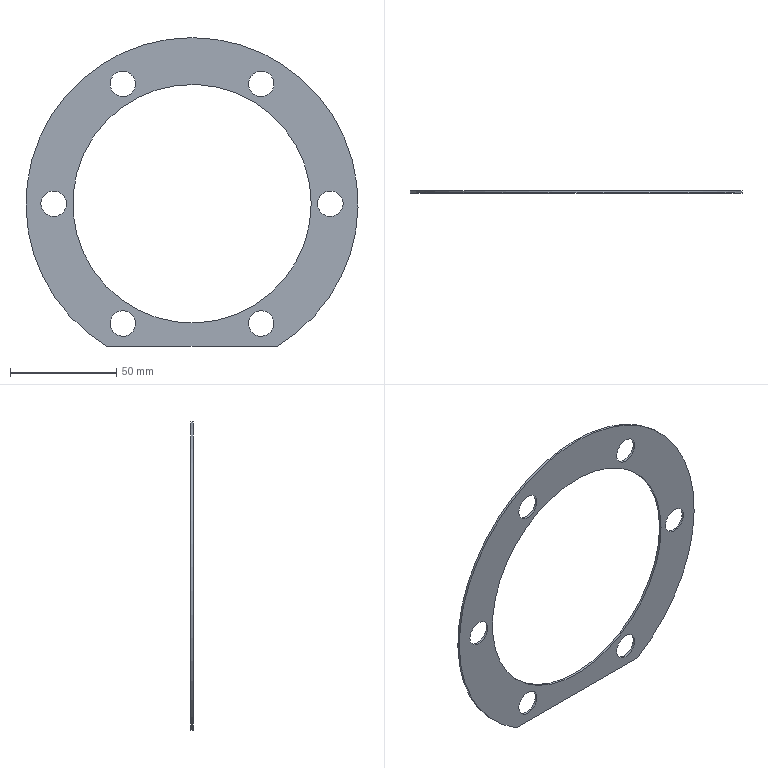Component | NX | T1_SHIM2_2 | 1 solid | 11 faces | box 156 x 1 x 145 mm | volume 7988 mm3 | cylinder 8 | plane 3 | commonest cylinder face diameters 12 x6 156 x1 112 x1
STEP:
#1=CARTESIAN_POINT('',(0.,0.,0.));
#2=DIRECTION('',(0.,0.,1.));
#3=DIRECTION('',(1.,0.,0.));
#4=AXIS2_PLACEMENT_3D('',#1,#2,#3);
#5=CARTESIAN_POINT('',(44.937,28.,198.5));
#6=VERTEX_POINT('',#5);
#7=CARTESIAN_POINT('',(-34.937,28.,198.5));
#8=VERTEX_POINT('',#7);
#9=CARTESIAN_POINT('',(5.,28.,265.5));
#10=DIRECTION('',(0.,-1.,0.));
#11=DIRECTION('',(1.,0.,0.));
#12=AXIS2_PLACEMENT_3D('',#9,#10,#11);
#13=CIRCLE('',#12,78.);
#14=CARTESIAN_POINT('',(5.,27.,265.5));
#15=DIRECTION('',(0.,1.,0.));
#16=DIRECTION('',(-1.,0.,0.));
#17=AXIS2_PLACEMENT_3D('',#14,#15,#16);
#18=CYLINDRICAL_SURFACE('',#17,78.);
#19=CARTESIAN_POINT('',(9.425,1.));
#20=DIRECTION('',(-1.,0.));
#21=VECTOR('',#20,1.);
#22=LINE('',#19,#21);
#23=(GEOMETRIC_REPRESENTATION_CONTEXT(2)PARAMETRIC_REPRESENTATION_CONTEXT()REPRESENTATION_CONTEXT('',''));
#24=DEFINITIONAL_REPRESENTATION('',(#22),#23);
#25=PCURVE('',#18,#24);
#26=CARTESIAN_POINT('',(5.,28.,265.5));
#27=DIRECTION('',(0.,-1.,0.));
#28=DIRECTION('',(1.,0.,0.));
#29=AXIS2_PLACEMENT_3D('',#26,#27,#28);
#30=PLANE('',#29);
#31=CARTESIAN_POINT('',(0.,0.));
#32=DIRECTION('',(1.,0.));
#33=AXIS2_PLACEMENT_2D('',#31,#32);
#34=CIRCLE('',#33,78.);
#35=(GEOMETRIC_REPRESENTATION_CONTEXT(2)PARAMETRIC_REPRESENTATION_CONTEXT()REPRESENTATION_CONTEXT('',''));
#36=DEFINITIONAL_REPRESENTATION('',(#34),#35);
#37=PCURVE('',#30,#36);
#38=SURFACE_CURVE('',#13,(#25,#37),.PCURVE_S1.);
#39=EDGE_CURVE('',#6,#8,#38,.T.);
#40=ORIENTED_EDGE('',*,*,#39,.T.);
#41=CARTESIAN_POINT('',(-34.937,27.,198.5));
#42=VERTEX_POINT('',#41);
#43=CARTESIAN_POINT('',(-34.937,27.,198.5));
#44=DIRECTION('',(0.,1.,0.));
#45=VECTOR('',#44,1.);
#46=LINE('',#43,#45);
#47=CARTESIAN_POINT('',(-1.033,0.));
#48=DIRECTION('',(0.,1.));
#49=VECTOR('',#48,1.);
#50=LINE('',#47,#49);
#51=(GEOMETRIC_REPRESENTATION_CONTEXT(2)PARAMETRIC_REPRESENTATION_CONTEXT()REPRESENTATION_CONTEXT('',''));
#52=DEFINITIONAL_REPRESENTATION('',(#50),#51);
#53=PCURVE('',#18,#52);
#54=CARTESIAN_POINT('',(-34.937,27.,198.5));
#55=DIRECTION('',(0.,0.,1.));
#56=DIRECTION('',(0.,-1.,0.));
#57=AXIS2_PLACEMENT_3D('',#54,#55,#56);
#58=PLANE('',#57);
#59=CARTESIAN_POINT('',(0.,0.));
#60=DIRECTION('',(-1.,0.));
#61=VECTOR('',#60,1.);
#62=LINE('',#59,#61);
#63=(GEOMETRIC_REPRESENTATION_CONTEXT(2)PARAMETRIC_REPRESENTATION_CONTEXT()REPRESENTATION_CONTEXT('',''));
#64=DEFINITIONAL_REPRESENTATION('',(#62),#63);
#65=PCURVE('',#58,#64);
#66=SURFACE_CURVE('',#46,(#53,#65),.PCURVE_S1.);
#67=EDGE_CURVE('',#42,#8,#66,.T.);
#68=ORIENTED_EDGE('',*,*,#67,.F.);
#69=CARTESIAN_POINT('',(44.937,27.,198.5));
#70=VERTEX_POINT('',#69);
#71=CARTESIAN_POINT('',(5.,27.,265.5));
#72=DIRECTION('',(0.,-1.,0.));
#73=DIRECTION('',(1.,0.,0.));
#74=AXIS2_PLACEMENT_3D('',#71,#72,#73);
#75=CIRCLE('',#74,78.);
#76=CARTESIAN_POINT('',(9.425,0.));
#77=DIRECTION('',(-1.,0.));
#78=VECTOR('',#77,1.);
#79=LINE('',#76,#78);
#80=(GEOMETRIC_REPRESENTATION_CONTEXT(2)PARAMETRIC_REPRESENTATION_CONTEXT()REPRESENTATION_CONTEXT('',''));
#81=DEFINITIONAL_REPRESENTATION('',(#79),#80);
#82=PCURVE('',#18,#81);
#83=CARTESIAN_POINT('',(5.,27.,265.5));
#84=DIRECTION('',(0.,-1.,0.));
#85=DIRECTION('',(1.,0.,0.));
#86=AXIS2_PLACEMENT_3D('',#83,#84,#85);
#87=PLANE('',#86);
#88=CARTESIAN_POINT('',(0.,0.));
#89=DIRECTION('',(1.,0.));
#90=AXIS2_PLACEMENT_2D('',#88,#89);
#91=CIRCLE('',#90,78.);
#92=(GEOMETRIC_REPRESENTATION_CONTEXT(2)PARAMETRIC_REPRESENTATION_CONTEXT()REPRESENTATION_CONTEXT('',''));
#93=DEFINITIONAL_REPRESENTATION('',(#91),#92);
#94=PCURVE('',#87,#93);
#95=SURFACE_CURVE('',#75,(#82,#94),.PCURVE_S1.);
#96=EDGE_CURVE('',#70,#42,#95,.T.);
#97=ORIENTED_EDGE('',*,*,#96,.F.);
#98=CARTESIAN_POINT('',(44.937,27.,198.5));
#99=DIRECTION('',(0.,-1.,0.));
#100=VECTOR('',#99,1.);
#101=LINE('',#98,#100);
#102=CARTESIAN_POINT('',(4.175,0.));
#103=DIRECTION('',(0.,-1.));
#104=VECTOR('',#103,1.);
#105=LINE('',#102,#104);
#106=(GEOMETRIC_REPRESENTATION_CONTEXT(2)PARAMETRIC_REPRESENTATION_CONTEXT()REPRESENTATION_CONTEXT('',''));
#107=DEFINITIONAL_REPRESENTATION('',(#105),#106);
#108=PCURVE('',#18,#107);
#109=CARTESIAN_POINT('',(0.,79.875));
#110=DIRECTION('',(1.,0.));
#111=VECTOR('',#110,1.);
#112=LINE('',#109,#111);
#113=(GEOMETRIC_REPRESENTATION_CONTEXT(2)PARAMETRIC_REPRESENTATION_CONTEXT()REPRESENTATION_CONTEXT('',''));
#114=DEFINITIONAL_REPRESENTATION('',(#112),#113);
#115=PCURVE('',#58,#114);
#116=SURFACE_CURVE('',#101,(#108,#115),.PCURVE_S1.);
#117=EDGE_CURVE('',#6,#70,#116,.T.);
#118=ORIENTED_EDGE('',*,*,#117,.F.);
#119=EDGE_LOOP('',(#40,#68,#97,#118));
#120=FACE_BOUND('',#119,.T.);
#121=ADVANCED_FACE('',(#120),#18,.T.);
#122=CARTESIAN_POINT('',(40.5,27.,326.988));
#123=VERTEX_POINT('',#122);
#124=CARTESIAN_POINT('',(37.5,27.,321.792));
#125=DIRECTION('',(0.,-1.,0.));
#126=DIRECTION('',(0.5,0.,0.866));
#127=AXIS2_PLACEMENT_3D('',#124,#125,#126);
#128=CIRCLE('',#127,6.);
#129=CARTESIAN_POINT('',(37.5,27.,321.792));
#130=DIRECTION('',(0.,1.,0.));
#131=DIRECTION('',(-1.,0.,0.));
#132=AXIS2_PLACEMENT_3D('',#129,#130,#131);
#133=CYLINDRICAL_SURFACE('',#132,6.);
#134=CARTESIAN_POINT('',(8.378,0.));
#135=DIRECTION('',(-1.,0.));
#136=VECTOR('',#135,1.);
#137=LINE('',#134,#136);
#138=(GEOMETRIC_REPRESENTATION_CONTEXT(2)PARAMETRIC_REPRESENTATION_CONTEXT()REPRESENTATION_CONTEXT('',''));
#139=DEFINITIONAL_REPRESENTATION('',(#137),#138);
#140=PCURVE('',#133,#139);
#141=CARTESIAN_POINT('',(32.5,56.292));
#142=DIRECTION('',(0.5,0.866));
#143=AXIS2_PLACEMENT_2D('',#141,#142);
#144=CIRCLE('',#143,6.);
#145=(GEOMETRIC_REPRESENTATION_CONTEXT(2)PARAMETRIC_REPRESENTATION_CONTEXT()REPRESENTATION_CONTEXT('',''));
#146=DEFINITIONAL_REPRESENTATION('',(#144),#145);
#147=PCURVE('',#87,#146);
#148=SURFACE_CURVE('',#128,(#140,#147),.PCURVE_S1.);
#149=EDGE_CURVE('',#123,#123,#148,.T.);
#150=ORIENTED_EDGE('',*,*,#149,.F.);
#151=CARTESIAN_POINT('',(40.5,28.,326.988));
#152=VERTEX_POINT('',#151);
#153=CARTESIAN_POINT('',(40.5,27.,326.988));
#154=CARTESIAN_POINT('',(40.5,28.,326.988));
#155=B_SPLINE_CURVE_WITH_KNOTS('',1,(#153,#154),.UNSPECIFIED.,.F.,.F.,(2,2),(0.,1.),.PIECEWISE_BEZIER_KNOTS.);
#156=CARTESIAN_POINT('',(8.378,0.));
#157=DIRECTION('',(0.,1.));
#158=VECTOR('',#157,1.);
#159=LINE('',#156,#158);
#160=(GEOMETRIC_REPRESENTATION_CONTEXT(2)PARAMETRIC_REPRESENTATION_CONTEXT()REPRESENTATION_CONTEXT('',''));
#161=DEFINITIONAL_REPRESENTATION('',(#159),#160);
#162=PCURVE('',#133,#161);
#163=CARTESIAN_POINT('',(2.094,0.));
#164=DIRECTION('',(0.,1.));
#165=VECTOR('',#164,1.);
#166=LINE('',#163,#165);
#167=(GEOMETRIC_REPRESENTATION_CONTEXT(2)PARAMETRIC_REPRESENTATION_CONTEXT()REPRESENTATION_CONTEXT('',''));
#168=DEFINITIONAL_REPRESENTATION('',(#166),#167);
#169=PCURVE('',#133,#168);
#170=SEAM_CURVE('',#155,(#162,#169),.PCURVE_S1.);
#171=EDGE_CURVE('',#123,#152,#170,.T.);
#172=ORIENTED_EDGE('',*,*,#171,.T.);
#173=CARTESIAN_POINT('',(37.5,28.,321.792));
#174=DIRECTION('',(0.,-1.,0.));
#175=DIRECTION('',(0.5,0.,0.866));
#176=AXIS2_PLACEMENT_3D('',#173,#174,#175);
#177=CIRCLE('',#176,6.);
#178=CARTESIAN_POINT('',(8.378,1.));
#179=DIRECTION('',(-1.,0.));
#180=VECTOR('',#179,1.);
#181=LINE('',#178,#180);
#182=(GEOMETRIC_REPRESENTATION_CONTEXT(2)PARAMETRIC_REPRESENTATION_CONTEXT()REPRESENTATION_CONTEXT('',''));
#183=DEFINITIONAL_REPRESENTATION('',(#181),#182);
#184=PCURVE('',#133,#183);
#185=CARTESIAN_POINT('',(32.5,56.292));
#186=DIRECTION('',(0.5,0.866));
#187=AXIS2_PLACEMENT_2D('',#185,#186);
#188=CIRCLE('',#187,6.);
#189=(GEOMETRIC_REPRESENTATION_CONTEXT(2)PARAMETRIC_REPRESENTATION_CONTEXT()REPRESENTATION_CONTEXT('',''));
#190=DEFINITIONAL_REPRESENTATION('',(#188),#189);
#191=PCURVE('',#30,#190);
#192=SURFACE_CURVE('',#177,(#184,#191),.PCURVE_S1.);
#193=EDGE_CURVE('',#152,#152,#192,.T.);
#194=ORIENTED_EDGE('',*,*,#193,.T.);
#195=ORIENTED_EDGE('',*,*,#171,.F.);
#196=EDGE_LOOP('',(#150,#172,#194,#195));
#197=FACE_BOUND('',#196,.F.);
#198=ADVANCED_FACE('',(#197),#133,.F.);
#199=CARTESIAN_POINT('',(40.5,27.,204.012));
#200=VERTEX_POINT('',#199);
#201=CARTESIAN_POINT('',(37.5,27.,209.208));
#202=DIRECTION('',(0.,-1.,0.));
#203=DIRECTION('',(0.5,0.,-0.866));
#204=AXIS2_PLACEMENT_3D('',#201,#202,#203);
#205=CIRCLE('',#204,6.);
#206=CARTESIAN_POINT('',(37.5,27.,209.208));
#207=DIRECTION('',(0.,1.,0.));
#208=DIRECTION('',(-1.,0.,0.));
#209=AXIS2_PLACEMENT_3D('',#206,#207,#208);
#210=CYLINDRICAL_SURFACE('',#209,6.);
#211=CARTESIAN_POINT('',(10.472,0.));
#212=DIRECTION('',(-1.,0.));
#213=VECTOR('',#212,1.);
#214=LINE('',#211,#213);
#215=(GEOMETRIC_REPRESENTATION_CONTEXT(2)PARAMETRIC_REPRESENTATION_CONTEXT()REPRESENTATION_CONTEXT('',''));
#216=DEFINITIONAL_REPRESENTATION('',(#214),#215);
#217=PCURVE('',#210,#216);
#218=CARTESIAN_POINT('',(32.5,-56.292));
#219=DIRECTION('',(0.5,-0.866));
#220=AXIS2_PLACEMENT_2D('',#218,#219);
#221=CIRCLE('',#220,6.);
#222=(GEOMETRIC_REPRESENTATION_CONTEXT(2)PARAMETRIC_REPRESENTATION_CONTEXT()REPRESENTATION_CONTEXT('',''));
#223=DEFINITIONAL_REPRESENTATION('',(#221),#222);
#224=PCURVE('',#87,#223);
#225=SURFACE_CURVE('',#205,(#217,#224),.PCURVE_S1.);
#226=EDGE_CURVE('',#200,#200,#225,.T.);
#227=ORIENTED_EDGE('',*,*,#226,.F.);
#228=CARTESIAN_POINT('',(40.5,28.,204.012));
#229=VERTEX_POINT('',#228);
#230=CARTESIAN_POINT('',(40.5,27.,204.012));
#231=CARTESIAN_POINT('',(40.5,28.,204.012));
#232=B_SPLINE_CURVE_WITH_KNOTS('',1,(#230,#231),.UNSPECIFIED.,.F.,.F.,(2,2),(0.,1.),.PIECEWISE_BEZIER_KNOTS.);
#233=CARTESIAN_POINT('',(10.472,0.));
#234=DIRECTION('',(0.,1.));
#235=VECTOR('',#234,1.);
#236=LINE('',#233,#235);
#237=(GEOMETRIC_REPRESENTATION_CONTEXT(2)PARAMETRIC_REPRESENTATION_CONTEXT()REPRESENTATION_CONTEXT('',''));
#238=DEFINITIONAL_REPRESENTATION('',(#236),#237);
#239=PCURVE('',#210,#238);
#240=CARTESIAN_POINT('',(4.189,0.));
#241=DIRECTION('',(0.,1.));
#242=VECTOR('',#241,1.);
#243=LINE('',#240,#242);
#244=(GEOMETRIC_REPRESENTATION_CONTEXT(2)PARAMETRIC_REPRESENTATION_CONTEXT()REPRESENTATION_CONTEXT('',''));
#245=DEFINITIONAL_REPRESENTATION('',(#243),#244);
#246=PCURVE('',#210,#245);
#247=SEAM_CURVE('',#232,(#239,#246),.PCURVE_S1.);
#248=EDGE_CURVE('',#200,#229,#247,.T.);
#249=ORIENTED_EDGE('',*,*,#248,.T.);
#250=CARTESIAN_POINT('',(37.5,28.,209.208));
#251=DIRECTION('',(0.,-1.,0.));
#252=DIRECTION('',(0.5,0.,-0.866));
#253=AXIS2_PLACEMENT_3D('',#250,#251,#252);
#254=CIRCLE('',#253,6.);
#255=CARTESIAN_POINT('',(10.472,1.));
#256=DIRECTION('',(-1.,0.));
#257=VECTOR('',#256,1.);
#258=LINE('',#255,#257);
#259=(GEOMETRIC_REPRESENTATION_CONTEXT(2)PARAMETRIC_REPRESENTATION_CONTEXT()REPRESENTATION_CONTEXT('',''));
#260=DEFINITIONAL_REPRESENTATION('',(#258),#259);
#261=PCURVE('',#210,#260);
#262=CARTESIAN_POINT('',(32.5,-56.292));
#263=DIRECTION('',(0.5,-0.866));
#264=AXIS2_PLACEMENT_2D('',#262,#263);
#265=CIRCLE('',#264,6.);
#266=(GEOMETRIC_REPRESENTATION_CONTEXT(2)PARAMETRIC_REPRESENTATION_CONTEXT()REPRESENTATION_CONTEXT('',''));
#267=DEFINITIONAL_REPRESENTATION('',(#265),#266);
#268=PCURVE('',#30,#267);
#269=SURFACE_CURVE('',#254,(#261,#268),.PCURVE_S1.);
#270=EDGE_CURVE('',#229,#229,#269,.T.);
#271=ORIENTED_EDGE('',*,*,#270,.T.);
#272=ORIENTED_EDGE('',*,*,#248,.F.);
#273=EDGE_LOOP('',(#227,#249,#271,#272));
#274=FACE_BOUND('',#273,.F.);
#275=ADVANCED_FACE('',(#274),#210,.F.);
#276=CARTESIAN_POINT('',(-30.5,27.,326.988));
#277=VERTEX_POINT('',#276);
#278=CARTESIAN_POINT('',(-27.5,27.,321.792));
#279=DIRECTION('',(0.,-1.,0.));
#280=DIRECTION('',(-0.5,0.,0.866));
#281=AXIS2_PLACEMENT_3D('',#278,#279,#280);
#282=CIRCLE('',#281,6.);
#283=CARTESIAN_POINT('',(-27.5,27.,321.792));
#284=DIRECTION('',(0.,1.,0.));
#285=DIRECTION('',(-1.,0.,0.));
#286=AXIS2_PLACEMENT_3D('',#283,#284,#285);
#287=CYLINDRICAL_SURFACE('',#286,6.);
#288=CARTESIAN_POINT('',(7.33,0.));
#289=DIRECTION('',(-1.,0.));
#290=VECTOR('',#289,1.);
#291=LINE('',#288,#290);
#292=(GEOMETRIC_REPRESENTATION_CONTEXT(2)PARAMETRIC_REPRESENTATION_CONTEXT()REPRESENTATION_CONTEXT('',''));
#293=DEFINITIONAL_REPRESENTATION('',(#291),#292);
#294=PCURVE('',#287,#293);
#295=CARTESIAN_POINT('',(-32.5,56.292));
#296=DIRECTION('',(-0.5,0.866));
#297=AXIS2_PLACEMENT_2D('',#295,#296);
#298=CIRCLE('',#297,6.);
#299=(GEOMETRIC_REPRESENTATION_CONTEXT(2)PARAMETRIC_REPRESENTATION_CONTEXT()REPRESENTATION_CONTEXT('',''));
#300=DEFINITIONAL_REPRESENTATION('',(#298),#299);
#301=PCURVE('',#87,#300);
#302=SURFACE_CURVE('',#282,(#294,#301),.PCURVE_S1.);
#303=EDGE_CURVE('',#277,#277,#302,.T.);
#304=ORIENTED_EDGE('',*,*,#303,.F.);
#305=CARTESIAN_POINT('',(-30.5,28.,326.988));
#306=VERTEX_POINT('',#305);
#307=CARTESIAN_POINT('',(-30.5,27.,326.988));
#308=CARTESIAN_POINT('',(-30.5,28.,326.988));
#309=B_SPLINE_CURVE_WITH_KNOTS('',1,(#307,#308),.UNSPECIFIED.,.F.,.F.,(2,2),(0.,1.),.PIECEWISE_BEZIER_KNOTS.);
#310=CARTESIAN_POINT('',(7.33,0.));
#311=DIRECTION('',(0.,1.));
#312=VECTOR('',#311,1.);
#313=LINE('',#310,#312);
#314=(GEOMETRIC_REPRESENTATION_CONTEXT(2)PARAMETRIC_REPRESENTATION_CONTEXT()REPRESENTATION_CONTEXT('',''));
#315=DEFINITIONAL_REPRESENTATION('',(#313),#314);
#316=PCURVE('',#287,#315);
#317=CARTESIAN_POINT('',(1.047,0.));
#318=DIRECTION('',(0.,1.));
#319=VECTOR('',#318,1.);
#320=LINE('',#317,#319);
#321=(GEOMETRIC_REPRESENTATION_CONTEXT(2)PARAMETRIC_REPRESENTATION_CONTEXT()REPRESENTATION_CONTEXT('',''));
#322=DEFINITIONAL_REPRESENTATION('',(#320),#321);
#323=PCURVE('',#287,#322);
#324=SEAM_CURVE('',#309,(#316,#323),.PCURVE_S1.);
#325=EDGE_CURVE('',#277,#306,#324,.T.);
#326=ORIENTED_EDGE('',*,*,#325,.T.);
#327=CARTESIAN_POINT('',(-27.5,28.,321.792));
#328=DIRECTION('',(0.,-1.,0.));
#329=DIRECTION('',(-0.5,0.,0.866));
#330=AXIS2_PLACEMENT_3D('',#327,#328,#329);
#331=CIRCLE('',#330,6.);
#332=CARTESIAN_POINT('',(7.33,1.));
#333=DIRECTION('',(-1.,0.));
#334=VECTOR('',#333,1.);
#335=LINE('',#332,#334);
#336=(GEOMETRIC_REPRESENTATION_CONTEXT(2)PARAMETRIC_REPRESENTATION_CONTEXT()REPRESENTATION_CONTEXT('',''));
#337=DEFINITIONAL_REPRESENTATION('',(#335),#336);
#338=PCURVE('',#287,#337);
#339=CARTESIAN_POINT('',(-32.5,56.292));
#340=DIRECTION('',(-0.5,0.866));
#341=AXIS2_PLACEMENT_2D('',#339,#340);
#342=CIRCLE('',#341,6.);
#343=(GEOMETRIC_REPRESENTATION_CONTEXT(2)PARAMETRIC_REPRESENTATION_CONTEXT()REPRESENTATION_CONTEXT('',''));
#344=DEFINITIONAL_REPRESENTATION('',(#342),#343);
#345=PCURVE('',#30,#344);
#346=SURFACE_CURVE('',#331,(#338,#345),.PCURVE_S1.);
#347=EDGE_CURVE('',#306,#306,#346,.T.);
#348=ORIENTED_EDGE('',*,*,#347,.T.);
#349=ORIENTED_EDGE('',*,*,#325,.F.);
#350=EDGE_LOOP('',(#304,#326,#348,#349));
#351=FACE_BOUND('',#350,.F.);
#352=ADVANCED_FACE('',(#351),#287,.F.);
#353=CARTESIAN_POINT('',(-30.5,27.,204.012));
#354=VERTEX_POINT('',#353);
#355=CARTESIAN_POINT('',(-27.5,27.,209.208));
#356=DIRECTION('',(0.,-1.,0.));
#357=DIRECTION('',(-0.5,0.,-0.866));
#358=AXIS2_PLACEMENT_3D('',#355,#356,#357);
#359=CIRCLE('',#358,6.);
#360=CARTESIAN_POINT('',(-27.5,27.,209.208));
#361=DIRECTION('',(0.,1.,0.));
#362=DIRECTION('',(-1.,0.,0.));
#363=AXIS2_PLACEMENT_3D('',#360,#361,#362);
#364=CYLINDRICAL_SURFACE('',#363,6.);
#365=CARTESIAN_POINT('',(11.519,0.));
#366=DIRECTION('',(-1.,0.));
#367=VECTOR('',#366,1.);
#368=LINE('',#365,#367);
#369=(GEOMETRIC_REPRESENTATION_CONTEXT(2)PARAMETRIC_REPRESENTATION_CONTEXT()REPRESENTATION_CONTEXT('',''));
#370=DEFINITIONAL_REPRESENTATION('',(#368),#369);
#371=PCURVE('',#364,#370);
#372=CARTESIAN_POINT('',(-32.5,-56.292));
#373=DIRECTION('',(-0.5,-0.866));
#374=AXIS2_PLACEMENT_2D('',#372,#373);
#375=CIRCLE('',#374,6.);
#376=(GEOMETRIC_REPRESENTATION_CONTEXT(2)PARAMETRIC_REPRESENTATION_CONTEXT()REPRESENTATION_CONTEXT('',''));
#377=DEFINITIONAL_REPRESENTATION('',(#375),#376);
#378=PCURVE('',#87,#377);
#379=SURFACE_CURVE('',#359,(#371,#378),.PCURVE_S1.);
#380=EDGE_CURVE('',#354,#354,#379,.T.);
#381=ORIENTED_EDGE('',*,*,#380,.F.);
#382=CARTESIAN_POINT('',(-30.5,28.,204.012));
#383=VERTEX_POINT('',#382);
#384=CARTESIAN_POINT('',(-30.5,27.,204.012));
#385=CARTESIAN_POINT('',(-30.5,28.,204.012));
#386=B_SPLINE_CURVE_WITH_KNOTS('',1,(#384,#385),.UNSPECIFIED.,.F.,.F.,(2,2),(0.,1.),.PIECEWISE_BEZIER_KNOTS.);
#387=CARTESIAN_POINT('',(11.519,0.));
#388=DIRECTION('',(0.,1.));
#389=VECTOR('',#388,1.);
#390=LINE('',#387,#389);
#391=(GEOMETRIC_REPRESENTATION_CONTEXT(2)PARAMETRIC_REPRESENTATION_CONTEXT()REPRESENTATION_CONTEXT('',''));
#392=DEFINITIONAL_REPRESENTATION('',(#390),#391);
#393=PCURVE('',#364,#392);
#394=CARTESIAN_POINT('',(5.236,0.));
#395=DIRECTION('',(0.,1.));
#396=VECTOR('',#395,1.);
#397=LINE('',#394,#396);
#398=(GEOMETRIC_REPRESENTATION_CONTEXT(2)PARAMETRIC_REPRESENTATION_CONTEXT()REPRESENTATION_CONTEXT('',''));
#399=DEFINITIONAL_REPRESENTATION('',(#397),#398);
#400=PCURVE('',#364,#399);
#401=SEAM_CURVE('',#386,(#393,#400),.PCURVE_S1.);
#402=EDGE_CURVE('',#354,#383,#401,.T.);
#403=ORIENTED_EDGE('',*,*,#402,.T.);
#404=CARTESIAN_POINT('',(-27.5,28.,209.208));
#405=DIRECTION('',(0.,-1.,0.));
#406=DIRECTION('',(-0.5,0.,-0.866));
#407=AXIS2_PLACEMENT_3D('',#404,#405,#406);
#408=CIRCLE('',#407,6.);
#409=CARTESIAN_POINT('',(11.519,1.));
#410=DIRECTION('',(-1.,0.));
#411=VECTOR('',#410,1.);
#412=LINE('',#409,#411);
#413=(GEOMETRIC_REPRESENTATION_CONTEXT(2)PARAMETRIC_REPRESENTATION_CONTEXT()REPRESENTATION_CONTEXT('',''));
#414=DEFINITIONAL_REPRESENTATION('',(#412),#413);
#415=PCURVE('',#364,#414);
#416=CARTESIAN_POINT('',(-32.5,-56.292));
#417=DIRECTION('',(-0.5,-0.866));
#418=AXIS2_PLACEMENT_2D('',#416,#417);
#419=CIRCLE('',#418,6.);
#420=(GEOMETRIC_REPRESENTATION_CONTEXT(2)PARAMETRIC_REPRESENTATION_CONTEXT()REPRESENTATION_CONTEXT('',''));
#421=DEFINITIONAL_REPRESENTATION('',(#419),#420);
#422=PCURVE('',#30,#421);
#423=SURFACE_CURVE('',#408,(#415,#422),.PCURVE_S1.);
#424=EDGE_CURVE('',#383,#383,#423,.T.);
#425=ORIENTED_EDGE('',*,*,#424,.T.);
#426=ORIENTED_EDGE('',*,*,#402,.F.);
#427=EDGE_LOOP('',(#381,#403,#425,#426));
#428=FACE_BOUND('',#427,.F.);
#429=ADVANCED_FACE('',(#428),#364,.F.);
#430=CARTESIAN_POINT('',(61.,27.,265.5));
#431=VERTEX_POINT('',#430);
#432=CARTESIAN_POINT('',(5.,27.,265.5));
#433=DIRECTION('',(0.,-1.,0.));
#434=DIRECTION('',(1.,0.,0.));
#435=AXIS2_PLACEMENT_3D('',#432,#433,#434);
#436=CIRCLE('',#435,56.);
#437=CARTESIAN_POINT('',(5.,27.,265.5));
#438=DIRECTION('',(0.,1.,0.));
#439=DIRECTION('',(-1.,0.,0.));
#440=AXIS2_PLACEMENT_3D('',#437,#438,#439);
#441=CYLINDRICAL_SURFACE('',#440,56.);
#442=CARTESIAN_POINT('',(9.425,0.));
#443=DIRECTION('',(-1.,0.));
#444=VECTOR('',#443,1.);
#445=LINE('',#442,#444);
#446=(GEOMETRIC_REPRESENTATION_CONTEXT(2)PARAMETRIC_REPRESENTATION_CONTEXT()REPRESENTATION_CONTEXT('',''));
#447=DEFINITIONAL_REPRESENTATION('',(#445),#446);
#448=PCURVE('',#441,#447);
#449=CARTESIAN_POINT('',(0.,0.));
#450=DIRECTION('',(1.,0.));
#451=AXIS2_PLACEMENT_2D('',#449,#450);
#452=CIRCLE('',#451,56.);
#453=(GEOMETRIC_REPRESENTATION_CONTEXT(2)PARAMETRIC_REPRESENTATION_CONTEXT()REPRESENTATION_CONTEXT('',''));
#454=DEFINITIONAL_REPRESENTATION('',(#452),#453);
#455=PCURVE('',#87,#454);
#456=SURFACE_CURVE('',#436,(#448,#455),.PCURVE_S1.);
#457=EDGE_CURVE('',#431,#431,#456,.T.);
#458=ORIENTED_EDGE('',*,*,#457,.F.);
#459=CARTESIAN_POINT('',(61.,28.,265.5));
#460=VERTEX_POINT('',#459);
#461=CARTESIAN_POINT('',(61.,27.,265.5));
#462=CARTESIAN_POINT('',(61.,28.,265.5));
#463=B_SPLINE_CURVE_WITH_KNOTS('',1,(#461,#462),.UNSPECIFIED.,.F.,.F.,(2,2),(0.,1.),.PIECEWISE_BEZIER_KNOTS.);
#464=CARTESIAN_POINT('',(9.425,0.));
#465=DIRECTION('',(0.,1.));
#466=VECTOR('',#465,1.);
#467=LINE('',#464,#466);
#468=(GEOMETRIC_REPRESENTATION_CONTEXT(2)PARAMETRIC_REPRESENTATION_CONTEXT()REPRESENTATION_CONTEXT('',''));
#469=DEFINITIONAL_REPRESENTATION('',(#467),#468);
#470=PCURVE('',#441,#469);
#471=CARTESIAN_POINT('',(3.142,0.));
#472=DIRECTION('',(0.,1.));
#473=VECTOR('',#472,1.);
#474=LINE('',#471,#473);
#475=(GEOMETRIC_REPRESENTATION_CONTEXT(2)PARAMETRIC_REPRESENTATION_CONTEXT()REPRESENTATION_CONTEXT('',''));
#476=DEFINITIONAL_REPRESENTATION('',(#474),#475);
#477=PCURVE('',#441,#476);
#478=SEAM_CURVE('',#463,(#470,#477),.PCURVE_S1.);
#479=EDGE_CURVE('',#431,#460,#478,.T.);
#480=ORIENTED_EDGE('',*,*,#479,.T.);
#481=CARTESIAN_POINT('',(5.,28.,265.5));
#482=DIRECTION('',(0.,-1.,0.));
#483=DIRECTION('',(1.,0.,0.));
#484=AXIS2_PLACEMENT_3D('',#481,#482,#483);
#485=CIRCLE('',#484,56.);
#486=CARTESIAN_POINT('',(9.425,1.));
#487=DIRECTION('',(-1.,0.));
#488=VECTOR('',#487,1.);
#489=LINE('',#486,#488);
#490=(GEOMETRIC_REPRESENTATION_CONTEXT(2)PARAMETRIC_REPRESENTATION_CONTEXT()REPRESENTATION_CONTEXT('',''));
#491=DEFINITIONAL_REPRESENTATION('',(#489),#490);
#492=PCURVE('',#441,#491);
#493=CARTESIAN_POINT('',(0.,0.));
#494=DIRECTION('',(1.,0.));
#495=AXIS2_PLACEMENT_2D('',#493,#494);
#496=CIRCLE('',#495,56.);
#497=(GEOMETRIC_REPRESENTATION_CONTEXT(2)PARAMETRIC_REPRESENTATION_CONTEXT()REPRESENTATION_CONTEXT('',''));
#498=DEFINITIONAL_REPRESENTATION('',(#496),#497);
#499=PCURVE('',#30,#498);
#500=SURFACE_CURVE('',#485,(#492,#499),.PCURVE_S1.);
#501=EDGE_CURVE('',#460,#460,#500,.T.);
#502=ORIENTED_EDGE('',*,*,#501,.T.);
#503=ORIENTED_EDGE('',*,*,#479,.F.);
#504=EDGE_LOOP('',(#458,#480,#502,#503));
#505=FACE_BOUND('',#504,.F.);
#506=ADVANCED_FACE('',(#505),#441,.F.);
#507=CARTESIAN_POINT('',(-66.,27.,265.5));
#508=VERTEX_POINT('',#507);
#509=CARTESIAN_POINT('',(-60.,27.,265.5));
#510=DIRECTION('',(0.,-1.,0.));
#511=DIRECTION('',(-1.,0.,0.));
#512=AXIS2_PLACEMENT_3D('',#509,#510,#511);
#513=CIRCLE('',#512,6.);
#514=CARTESIAN_POINT('',(-60.,27.,265.5));
#515=DIRECTION('',(0.,1.,0.));
#516=DIRECTION('',(-1.,0.,0.));
#517=AXIS2_PLACEMENT_3D('',#514,#515,#516);
#518=CYLINDRICAL_SURFACE('',#517,6.);
#519=CARTESIAN_POINT('',(6.283,0.));
#520=DIRECTION('',(-1.,0.));
#521=VECTOR('',#520,1.);
#522=LINE('',#519,#521);
#523=(GEOMETRIC_REPRESENTATION_CONTEXT(2)PARAMETRIC_REPRESENTATION_CONTEXT()REPRESENTATION_CONTEXT('',''));
#524=DEFINITIONAL_REPRESENTATION('',(#522),#523);
#525=PCURVE('',#518,#524);
#526=CARTESIAN_POINT('',(-65.,0.));
#527=DIRECTION('',(-1.,0.));
#528=AXIS2_PLACEMENT_2D('',#526,#527);
#529=CIRCLE('',#528,6.);
#530=(GEOMETRIC_REPRESENTATION_CONTEXT(2)PARAMETRIC_REPRESENTATION_CONTEXT()REPRESENTATION_CONTEXT('',''));
#531=DEFINITIONAL_REPRESENTATION('',(#529),#530);
#532=PCURVE('',#87,#531);
#533=SURFACE_CURVE('',#513,(#525,#532),.PCURVE_S1.);
#534=EDGE_CURVE('',#508,#508,#533,.T.);
#535=ORIENTED_EDGE('',*,*,#534,.F.);
#536=CARTESIAN_POINT('',(-66.,28.,265.5));
#537=VERTEX_POINT('',#536);
#538=CARTESIAN_POINT('',(-66.,27.,265.5));
#539=CARTESIAN_POINT('',(-66.,28.,265.5));
#540=B_SPLINE_CURVE_WITH_KNOTS('',1,(#538,#539),.UNSPECIFIED.,.F.,.F.,(2,2),(0.,1.),.PIECEWISE_BEZIER_KNOTS.);
#541=CARTESIAN_POINT('',(6.283,0.));
#542=DIRECTION('',(0.,1.));
#543=VECTOR('',#542,1.);
#544=LINE('',#541,#543);
#545=(GEOMETRIC_REPRESENTATION_CONTEXT(2)PARAMETRIC_REPRESENTATION_CONTEXT()REPRESENTATION_CONTEXT('',''));
#546=DEFINITIONAL_REPRESENTATION('',(#544),#545);
#547=PCURVE('',#518,#546);
#548=CARTESIAN_POINT('',(0.,0.));
#549=DIRECTION('',(0.,1.));
#550=VECTOR('',#549,1.);
#551=LINE('',#548,#550);
#552=(GEOMETRIC_REPRESENTATION_CONTEXT(2)PARAMETRIC_REPRESENTATION_CONTEXT()REPRESENTATION_CONTEXT('',''));
#553=DEFINITIONAL_REPRESENTATION('',(#551),#552);
#554=PCURVE('',#518,#553);
#555=SEAM_CURVE('',#540,(#547,#554),.PCURVE_S1.);
#556=EDGE_CURVE('',#508,#537,#555,.T.);
#557=ORIENTED_EDGE('',*,*,#556,.T.);
#558=CARTESIAN_POINT('',(-60.,28.,265.5));
#559=DIRECTION('',(0.,-1.,0.));
#560=DIRECTION('',(-1.,0.,0.));
#561=AXIS2_PLACEMENT_3D('',#558,#559,#560);
#562=CIRCLE('',#561,6.);
#563=CARTESIAN_POINT('',(6.283,1.));
#564=DIRECTION('',(-1.,0.));
#565=VECTOR('',#564,1.);
#566=LINE('',#563,#565);
#567=(GEOMETRIC_REPRESENTATION_CONTEXT(2)PARAMETRIC_REPRESENTATION_CONTEXT()REPRESENTATION_CONTEXT('',''));
#568=DEFINITIONAL_REPRESENTATION('',(#566),#567);
#569=PCURVE('',#518,#568);
#570=CARTESIAN_POINT('',(-65.,0.));
#571=DIRECTION('',(-1.,0.));
#572=AXIS2_PLACEMENT_2D('',#570,#571);
#573=CIRCLE('',#572,6.);
#574=(GEOMETRIC_REPRESENTATION_CONTEXT(2)PARAMETRIC_REPRESENTATION_CONTEXT()REPRESENTATION_CONTEXT('',''));
#575=DEFINITIONAL_REPRESENTATION('',(#573),#574);
#576=PCURVE('',#30,#575);
#577=SURFACE_CURVE('',#562,(#569,#576),.PCURVE_S1.);
#578=EDGE_CURVE('',#537,#537,#577,.T.);
#579=ORIENTED_EDGE('',*,*,#578,.T.);
#580=ORIENTED_EDGE('',*,*,#556,.F.);
#581=EDGE_LOOP('',(#535,#557,#579,#580));
#582=FACE_BOUND('',#581,.F.);
#583=ADVANCED_FACE('',(#582),#518,.F.);
#584=CARTESIAN_POINT('',(-34.937,28.,198.5));
#585=DIRECTION('',(1.,0.,0.));
#586=VECTOR('',#585,1.);
#587=LINE('',#584,#586);
#588=CARTESIAN_POINT('',(-1.,0.));
#589=DIRECTION('',(0.,1.));
#590=VECTOR('',#589,1.);
#591=LINE('',#588,#590);
#592=(GEOMETRIC_REPRESENTATION_CONTEXT(2)PARAMETRIC_REPRESENTATION_CONTEXT()REPRESENTATION_CONTEXT('',''));
#593=DEFINITIONAL_REPRESENTATION('',(#591),#592);
#594=PCURVE('',#58,#593);
#595=CARTESIAN_POINT('',(-39.937,-67.));
#596=DIRECTION('',(1.,0.));
#597=VECTOR('',#596,1.);
#598=LINE('',#595,#597);
#599=(GEOMETRIC_REPRESENTATION_CONTEXT(2)PARAMETRIC_REPRESENTATION_CONTEXT()REPRESENTATION_CONTEXT('',''));
#600=DEFINITIONAL_REPRESENTATION('',(#598),#599);
#601=PCURVE('',#30,#600);
#602=SURFACE_CURVE('',#587,(#594,#601),.PCURVE_S1.);
#603=EDGE_CURVE('',#8,#6,#602,.T.);
#604=ORIENTED_EDGE('',*,*,#603,.T.);
#605=ORIENTED_EDGE('',*,*,#117,.T.);
#606=CARTESIAN_POINT('',(-34.937,27.,198.5));
#607=DIRECTION('',(1.,0.,0.));
#608=VECTOR('',#607,1.);
#609=LINE('',#606,#608);
#610=CARTESIAN_POINT('',(0.,0.));
#611=DIRECTION('',(0.,1.));
#612=VECTOR('',#611,1.);
#613=LINE('',#610,#612);
#614=(GEOMETRIC_REPRESENTATION_CONTEXT(2)PARAMETRIC_REPRESENTATION_CONTEXT()REPRESENTATION_CONTEXT('',''));
#615=DEFINITIONAL_REPRESENTATION('',(#613),#614);
#616=PCURVE('',#58,#615);
#617=CARTESIAN_POINT('',(-39.937,-67.));
#618=DIRECTION('',(1.,0.));
#619=VECTOR('',#618,1.);
#620=LINE('',#617,#619);
#621=(GEOMETRIC_REPRESENTATION_CONTEXT(2)PARAMETRIC_REPRESENTATION_CONTEXT()REPRESENTATION_CONTEXT('',''));
#622=DEFINITIONAL_REPRESENTATION('',(#620),#621);
#623=PCURVE('',#87,#622);
#624=SURFACE_CURVE('',#609,(#616,#623),.PCURVE_S1.);
#625=EDGE_CURVE('',#42,#70,#624,.T.);
#626=ORIENTED_EDGE('',*,*,#625,.F.);
#627=ORIENTED_EDGE('',*,*,#67,.T.);
#628=EDGE_LOOP('',(#604,#605,#626,#627));
#629=FACE_BOUND('',#628,.T.);
#630=ADVANCED_FACE('',(#629),#58,.F.);
#631=CARTESIAN_POINT('',(76.,27.,265.5));
#632=VERTEX_POINT('',#631);
#633=CARTESIAN_POINT('',(70.,27.,265.5));
#634=DIRECTION('',(0.,-1.,0.));
#635=DIRECTION('',(1.,0.,0.));
#636=AXIS2_PLACEMENT_3D('',#633,#634,#635);
#637=CIRCLE('',#636,6.);
#638=CARTESIAN_POINT('',(70.,27.,265.5));
#639=DIRECTION('',(0.,1.,0.));
#640=DIRECTION('',(-1.,0.,0.));
#641=AXIS2_PLACEMENT_3D('',#638,#639,#640);
#642=CYLINDRICAL_SURFACE('',#641,6.);
#643=CARTESIAN_POINT('',(9.425,0.));
#644=DIRECTION('',(-1.,0.));
#645=VECTOR('',#644,1.);
#646=LINE('',#643,#645);
#647=(GEOMETRIC_REPRESENTATION_CONTEXT(2)PARAMETRIC_REPRESENTATION_CONTEXT()REPRESENTATION_CONTEXT('',''));
#648=DEFINITIONAL_REPRESENTATION('',(#646),#647);
#649=PCURVE('',#642,#648);
#650=CARTESIAN_POINT('',(65.,0.));
#651=DIRECTION('',(1.,0.));
#652=AXIS2_PLACEMENT_2D('',#650,#651);
#653=CIRCLE('',#652,6.);
#654=(GEOMETRIC_REPRESENTATION_CONTEXT(2)PARAMETRIC_REPRESENTATION_CONTEXT()REPRESENTATION_CONTEXT('',''));
#655=DEFINITIONAL_REPRESENTATION('',(#653),#654);
#656=PCURVE('',#87,#655);
#657=SURFACE_CURVE('',#637,(#649,#656),.PCURVE_S1.);
#658=EDGE_CURVE('',#632,#632,#657,.T.);
#659=ORIENTED_EDGE('',*,*,#658,.F.);
#660=CARTESIAN_POINT('',(76.,28.,265.5));
#661=VERTEX_POINT('',#660);
#662=CARTESIAN_POINT('',(76.,27.,265.5));
#663=CARTESIAN_POINT('',(76.,28.,265.5));
#664=B_SPLINE_CURVE_WITH_KNOTS('',1,(#662,#663),.UNSPECIFIED.,.F.,.F.,(2,2),(0.,1.),.PIECEWISE_BEZIER_KNOTS.);
#665=CARTESIAN_POINT('',(9.425,0.));
#666=DIRECTION('',(0.,1.));
#667=VECTOR('',#666,1.);
#668=LINE('',#665,#667);
#669=(GEOMETRIC_REPRESENTATION_CONTEXT(2)PARAMETRIC_REPRESENTATION_CONTEXT()REPRESENTATION_CONTEXT('',''));
#670=DEFINITIONAL_REPRESENTATION('',(#668),#669);
#671=PCURVE('',#642,#670);
#672=CARTESIAN_POINT('',(3.142,0.));
#673=DIRECTION('',(0.,1.));
#674=VECTOR('',#673,1.);
#675=LINE('',#672,#674);
#676=(GEOMETRIC_REPRESENTATION_CONTEXT(2)PARAMETRIC_REPRESENTATION_CONTEXT()REPRESENTATION_CONTEXT('',''));
#677=DEFINITIONAL_REPRESENTATION('',(#675),#676);
#678=PCURVE('',#642,#677);
#679=SEAM_CURVE('',#664,(#671,#678),.PCURVE_S1.);
#680=EDGE_CURVE('',#632,#661,#679,.T.);
#681=ORIENTED_EDGE('',*,*,#680,.T.);
#682=CARTESIAN_POINT('',(70.,28.,265.5));
#683=DIRECTION('',(0.,-1.,0.));
#684=DIRECTION('',(1.,0.,0.));
#685=AXIS2_PLACEMENT_3D('',#682,#683,#684);
#686=CIRCLE('',#685,6.);
#687=CARTESIAN_POINT('',(9.425,1.));
#688=DIRECTION('',(-1.,0.));
#689=VECTOR('',#688,1.);
#690=LINE('',#687,#689);
#691=(GEOMETRIC_REPRESENTATION_CONTEXT(2)PARAMETRIC_REPRESENTATION_CONTEXT()REPRESENTATION_CONTEXT('',''));
#692=DEFINITIONAL_REPRESENTATION('',(#690),#691);
#693=PCURVE('',#642,#692);
#694=CARTESIAN_POINT('',(65.,0.));
#695=DIRECTION('',(1.,0.));
#696=AXIS2_PLACEMENT_2D('',#694,#695);
#697=CIRCLE('',#696,6.);
#698=(GEOMETRIC_REPRESENTATION_CONTEXT(2)PARAMETRIC_REPRESENTATION_CONTEXT()REPRESENTATION_CONTEXT('',''));
#699=DEFINITIONAL_REPRESENTATION('',(#697),#698);
#700=PCURVE('',#30,#699);
#701=SURFACE_CURVE('',#686,(#693,#700),.PCURVE_S1.);
#702=EDGE_CURVE('',#661,#661,#701,.T.);
#703=ORIENTED_EDGE('',*,*,#702,.T.);
#704=ORIENTED_EDGE('',*,*,#680,.F.);
#705=EDGE_LOOP('',(#659,#681,#703,#704));
#706=FACE_BOUND('',#705,.F.);
#707=ADVANCED_FACE('',(#706),#642,.F.);
#708=ORIENTED_EDGE('',*,*,#96,.T.);
#709=ORIENTED_EDGE('',*,*,#625,.T.);
#710=EDGE_LOOP('',(#708,#709));
#711=FACE_BOUND('',#710,.T.);
#712=ORIENTED_EDGE('',*,*,#534,.F.);
#713=EDGE_LOOP('',(#712));
#714=FACE_BOUND('',#713,.T.);
#715=ORIENTED_EDGE('',*,*,#457,.F.);
#716=EDGE_LOOP('',(#715));
#717=FACE_BOUND('',#716,.T.);
#718=ORIENTED_EDGE('',*,*,#380,.F.);
#719=EDGE_LOOP('',(#718));
#720=FACE_BOUND('',#719,.T.);
#721=ORIENTED_EDGE('',*,*,#303,.F.);
#722=EDGE_LOOP('',(#721));
#723=FACE_BOUND('',#722,.T.);
#724=ORIENTED_EDGE('',*,*,#226,.F.);
#725=EDGE_LOOP('',(#724));
#726=FACE_BOUND('',#725,.T.);
#727=ORIENTED_EDGE('',*,*,#149,.F.);
#728=EDGE_LOOP('',(#727));
#729=FACE_BOUND('',#728,.T.);
#730=ORIENTED_EDGE('',*,*,#658,.F.);
#731=EDGE_LOOP('',(#730));
#732=FACE_BOUND('',#731,.T.);
#733=ADVANCED_FACE('',(#711,#714,#717,#720,#723,#726,#729,#732),#87,.T.);
#734=ORIENTED_EDGE('',*,*,#39,.F.);
#735=ORIENTED_EDGE('',*,*,#603,.F.);
#736=EDGE_LOOP('',(#734,#735));
#737=FACE_BOUND('',#736,.T.);
#738=ORIENTED_EDGE('',*,*,#578,.T.);
#739=EDGE_LOOP('',(#738));
#740=FACE_BOUND('',#739,.T.);
#741=ORIENTED_EDGE('',*,*,#501,.T.);
#742=EDGE_LOOP('',(#741));
#743=FACE_BOUND('',#742,.T.);
#744=ORIENTED_EDGE('',*,*,#424,.T.);
#745=EDGE_LOOP('',(#744));
#746=FACE_BOUND('',#745,.T.);
#747=ORIENTED_EDGE('',*,*,#347,.T.);
#748=EDGE_LOOP('',(#747));
#749=FACE_BOUND('',#748,.T.);
#750=ORIENTED_EDGE('',*,*,#270,.T.);
#751=EDGE_LOOP('',(#750));
#752=FACE_BOUND('',#751,.T.);
#753=ORIENTED_EDGE('',*,*,#193,.T.);
#754=EDGE_LOOP('',(#753));
#755=FACE_BOUND('',#754,.T.);
#756=ORIENTED_EDGE('',*,*,#702,.T.);
#757=EDGE_LOOP('',(#756));
#758=FACE_BOUND('',#757,.T.);
#759=ADVANCED_FACE('',(#737,#740,#743,#746,#749,#752,#755,#758),#30,.F.);
#760=CLOSED_SHELL('',(#121,#198,#275,#352,#429,#506,#583,#630,#707,#733,#759));
#761=MANIFOLD_SOLID_BREP('',#760);
#762=(LENGTH_UNIT()NAMED_UNIT(*)SI_UNIT(.MILLI.,.METRE.));
#763=UNCERTAINTY_MEASURE_WITH_UNIT(LENGTH_MEASURE(0.000005),#762,'','');
#764=(NAMED_UNIT(*)PLANE_ANGLE_UNIT()SI_UNIT($,.RADIAN.));
#765=(NAMED_UNIT(*)SI_UNIT($,.STERADIAN.)SOLID_ANGLE_UNIT());
#766=(GEOMETRIC_REPRESENTATION_CONTEXT(3)GLOBAL_UNCERTAINTY_ASSIGNED_CONTEXT((#763))GLOBAL_UNIT_ASSIGNED_CONTEXT((#762,#764,#765))REPRESENTATION_CONTEXT('',''));
#767=ADVANCED_BREP_SHAPE_REPRESENTATION('',(#4,#761),#766);